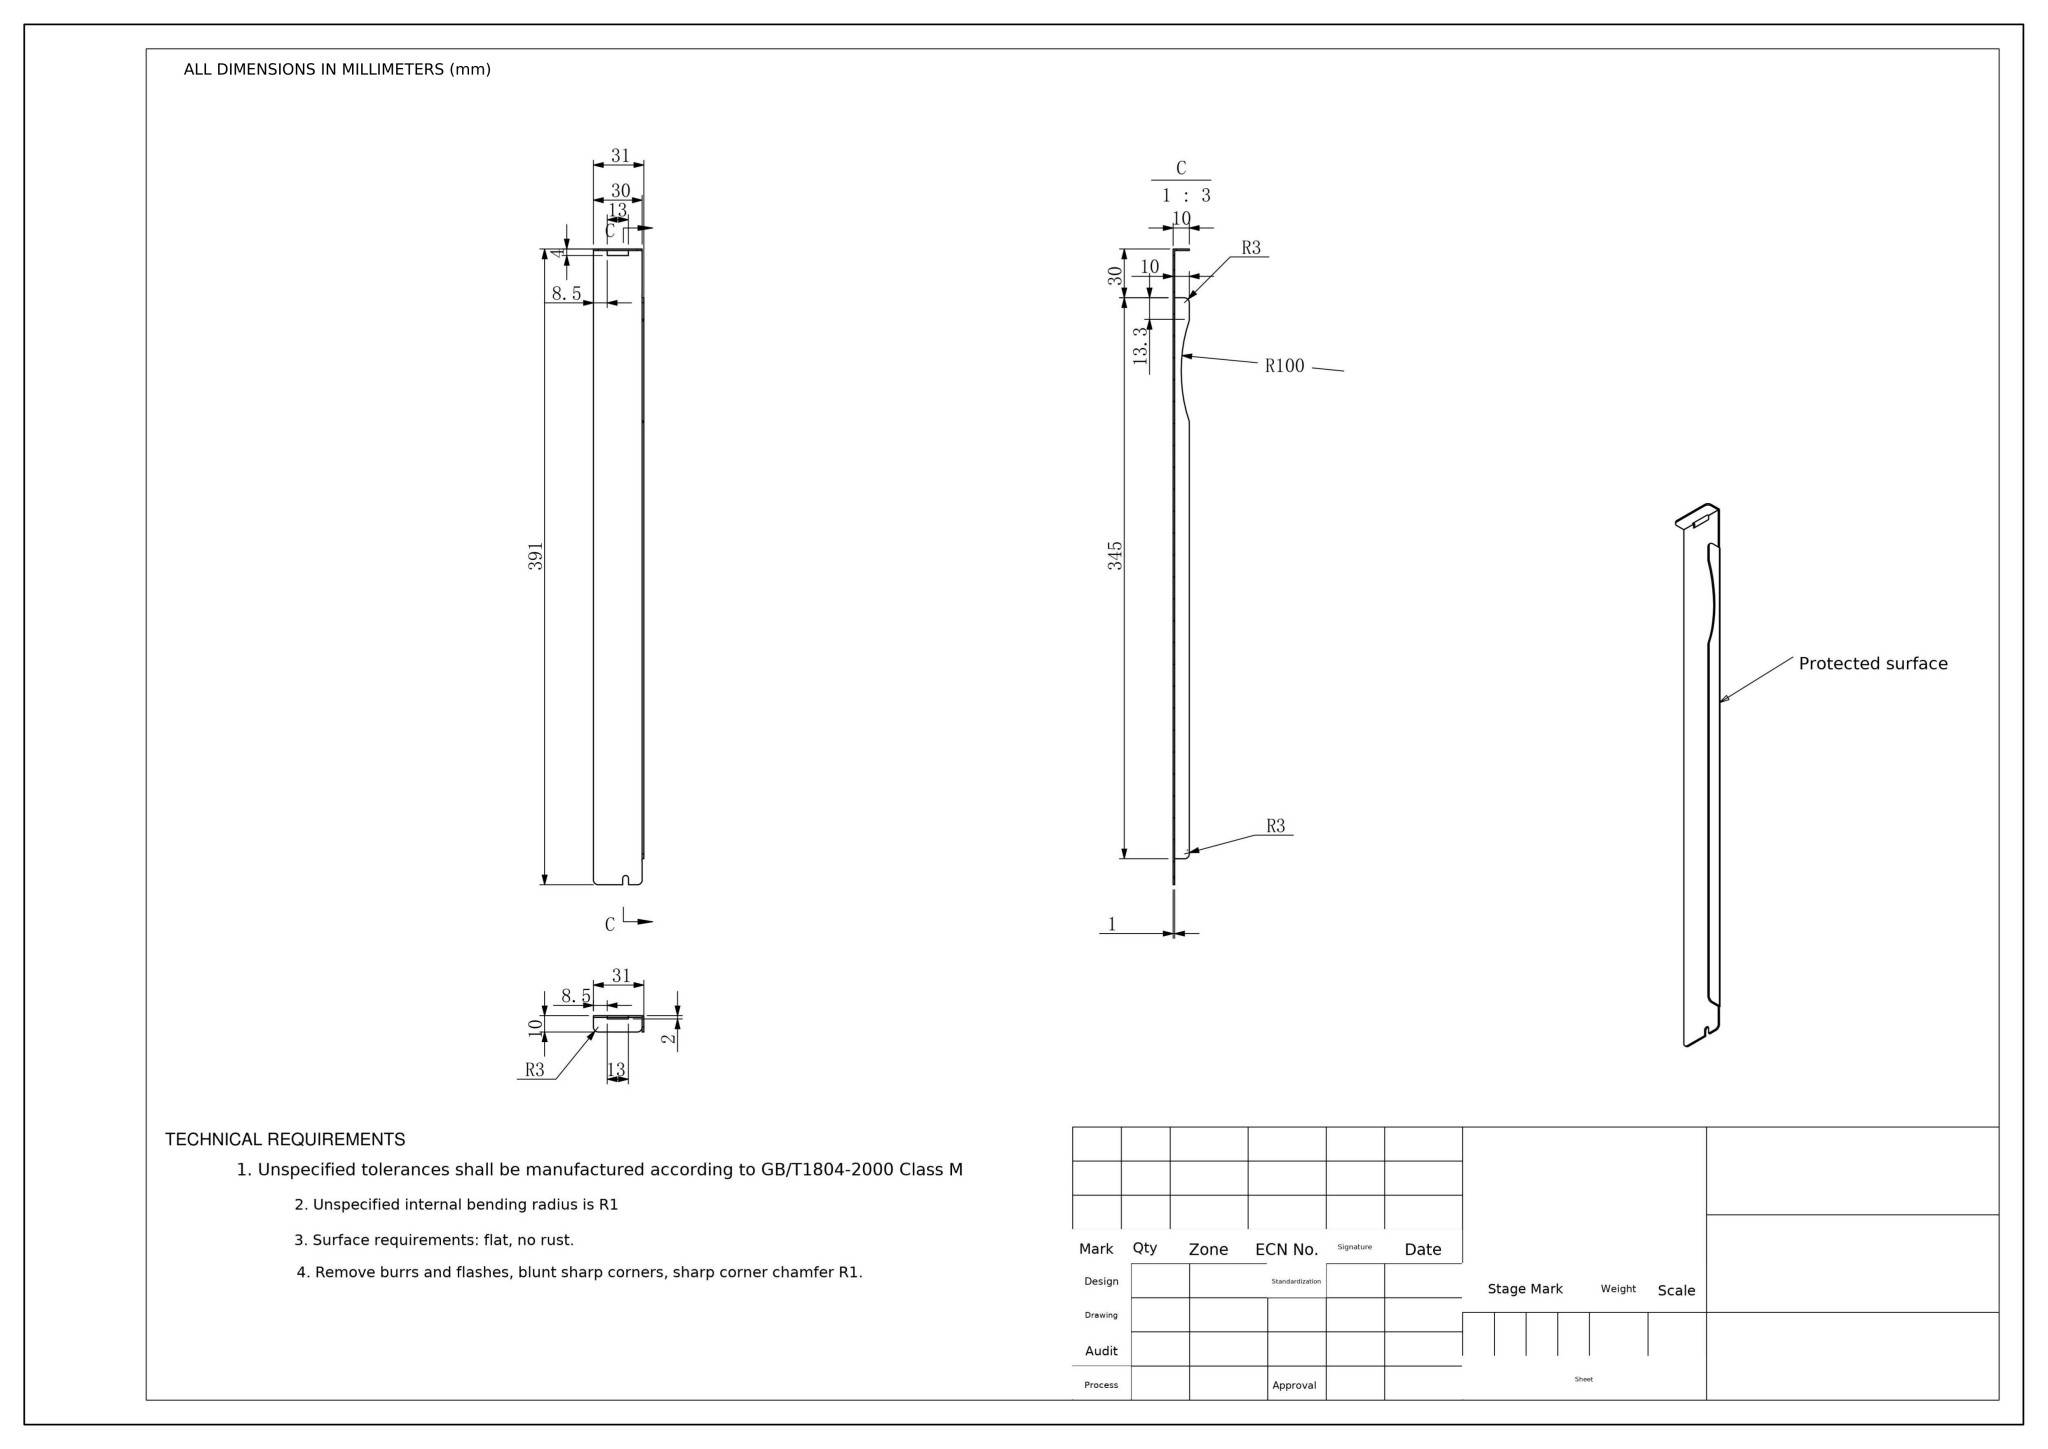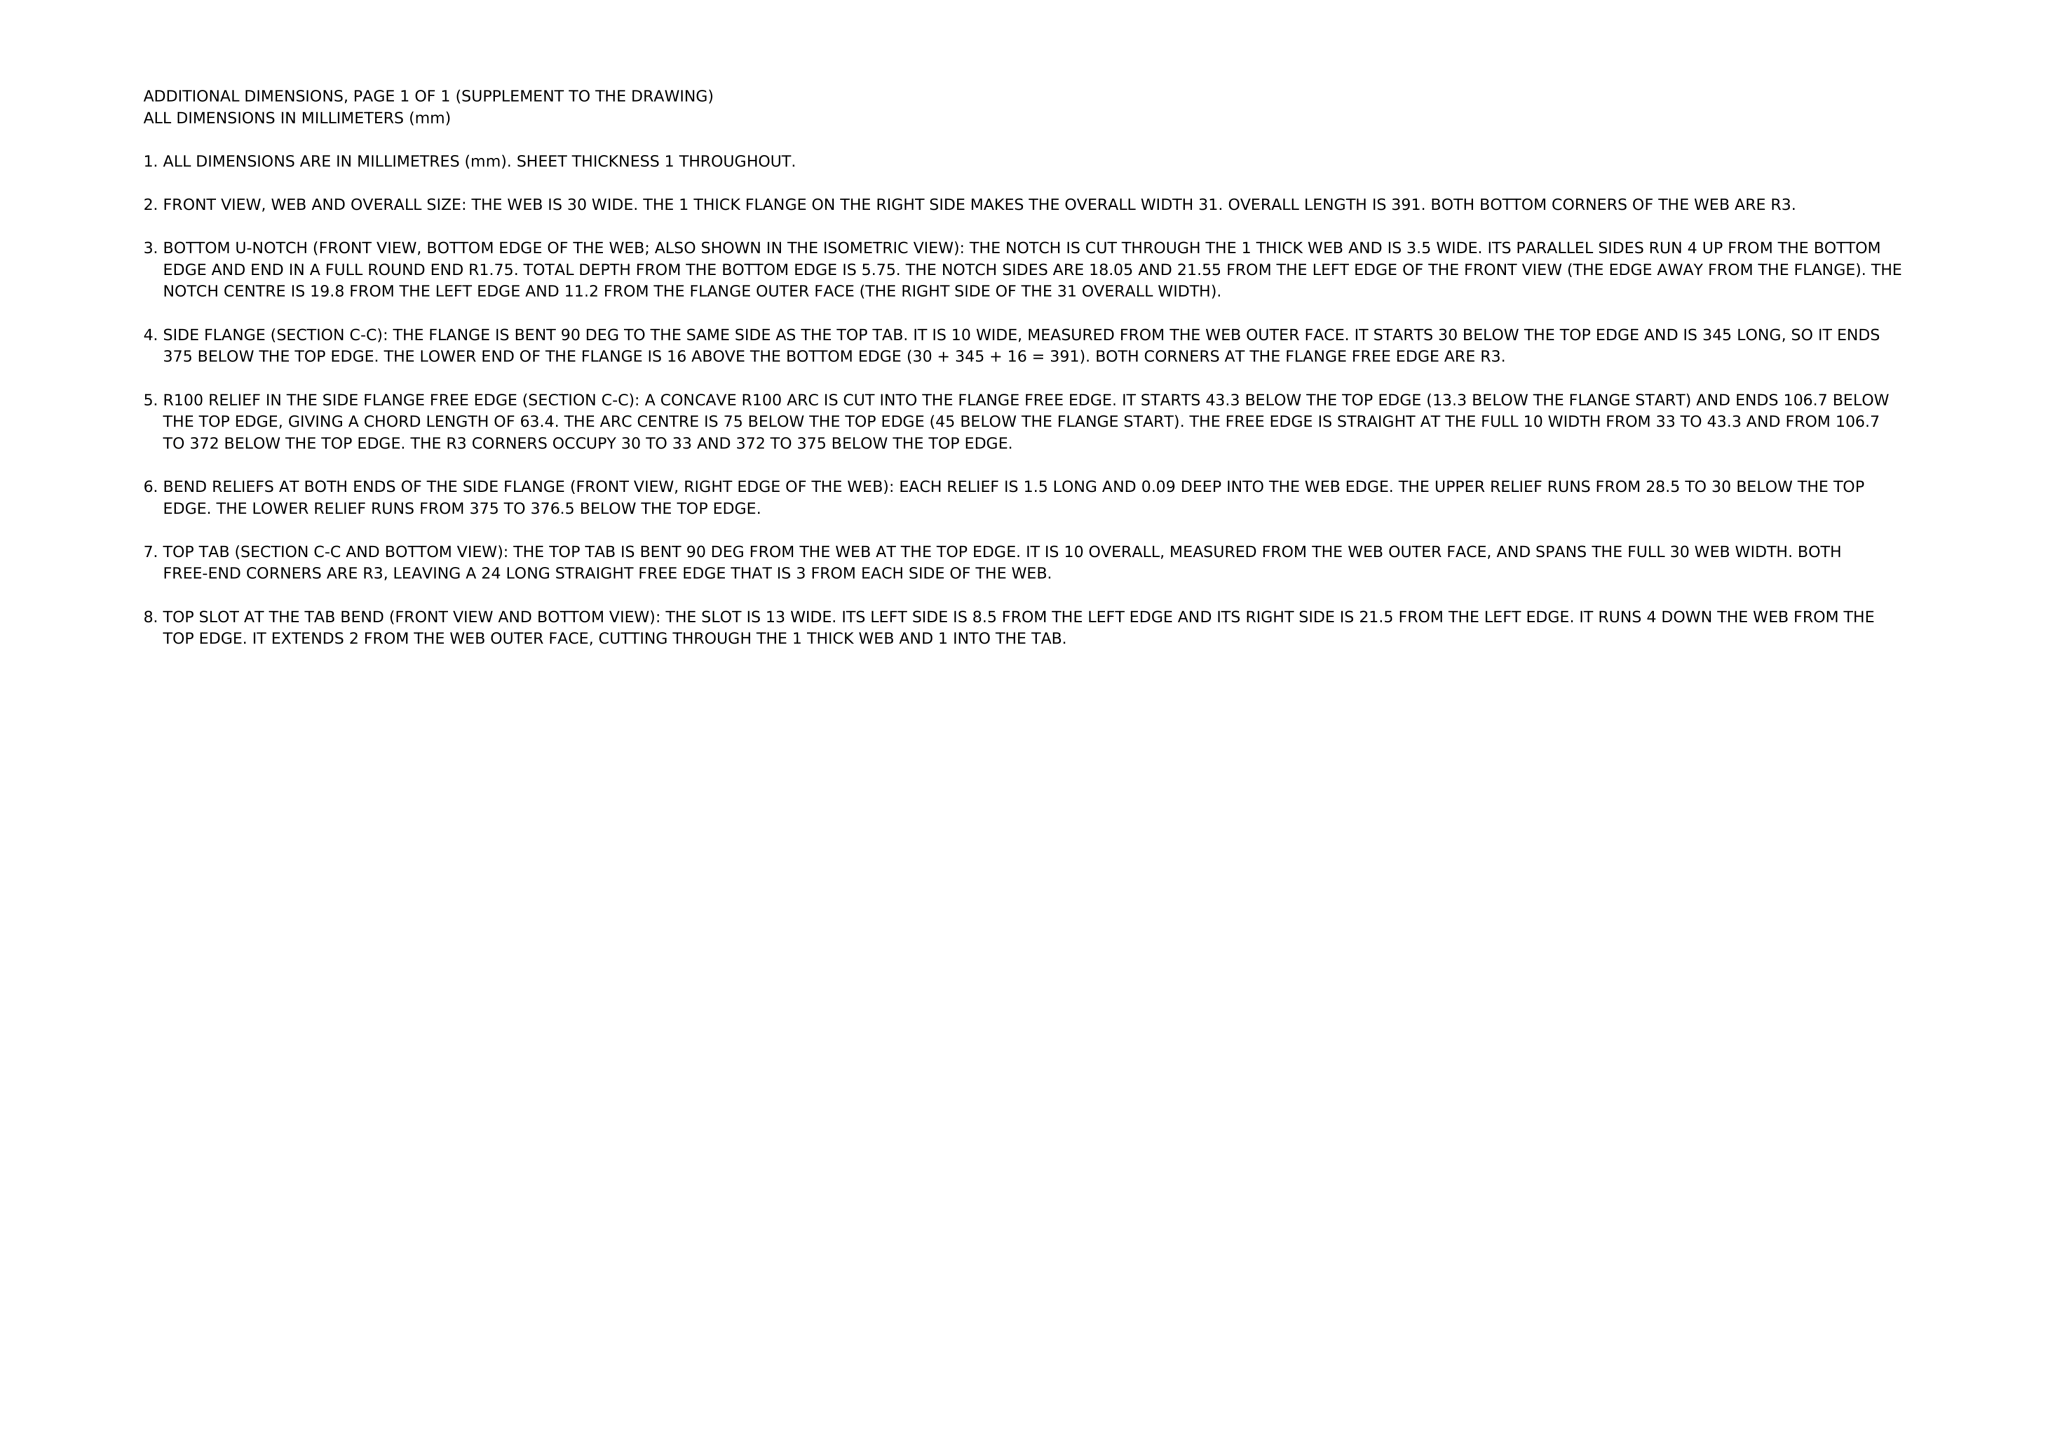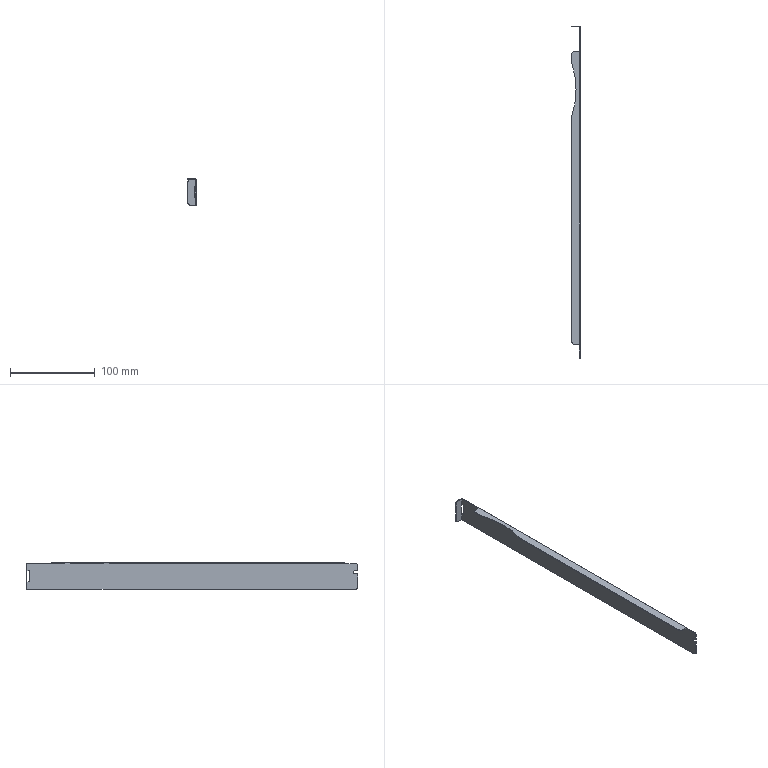Part | NX | mm | 1 solid | 50 faces | box 10 x 391 x 31 mm | volume 15067 mm3 | plane 30 | cylinder 20 | commonest cylinder face diameters 6 x8 2.004 x5 0.004 x5 3.5 x1 200 x1